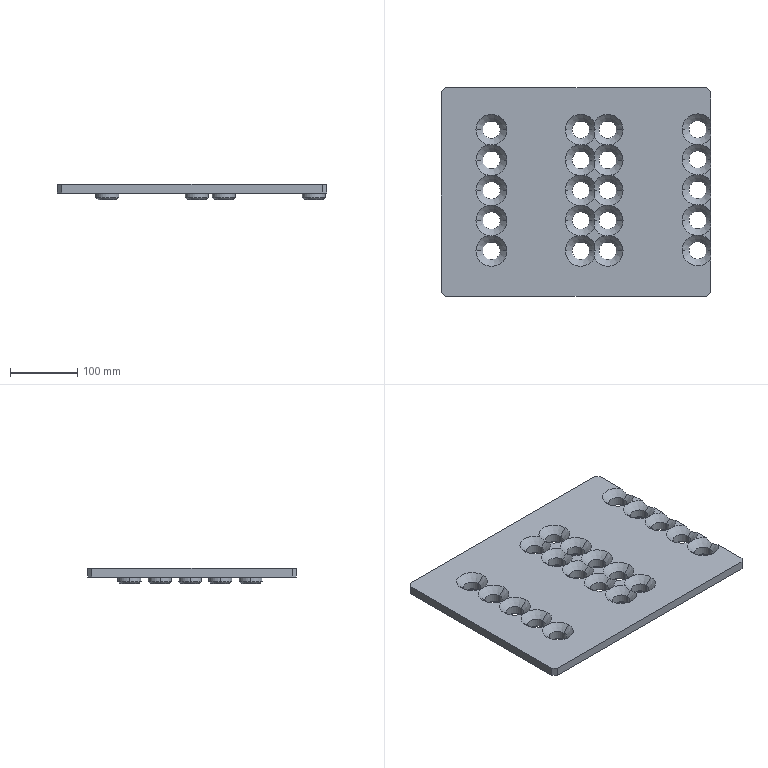Component | SolidWorks | AD12-SquareCellPressPlate.SDPRT-1 | 1 solid | 214 faces | volume 1431438 mm3 | cone 88 | cylinder 88 | plane 38 | commonest cylinder face diameters 34 x40 26 x40 22 x8